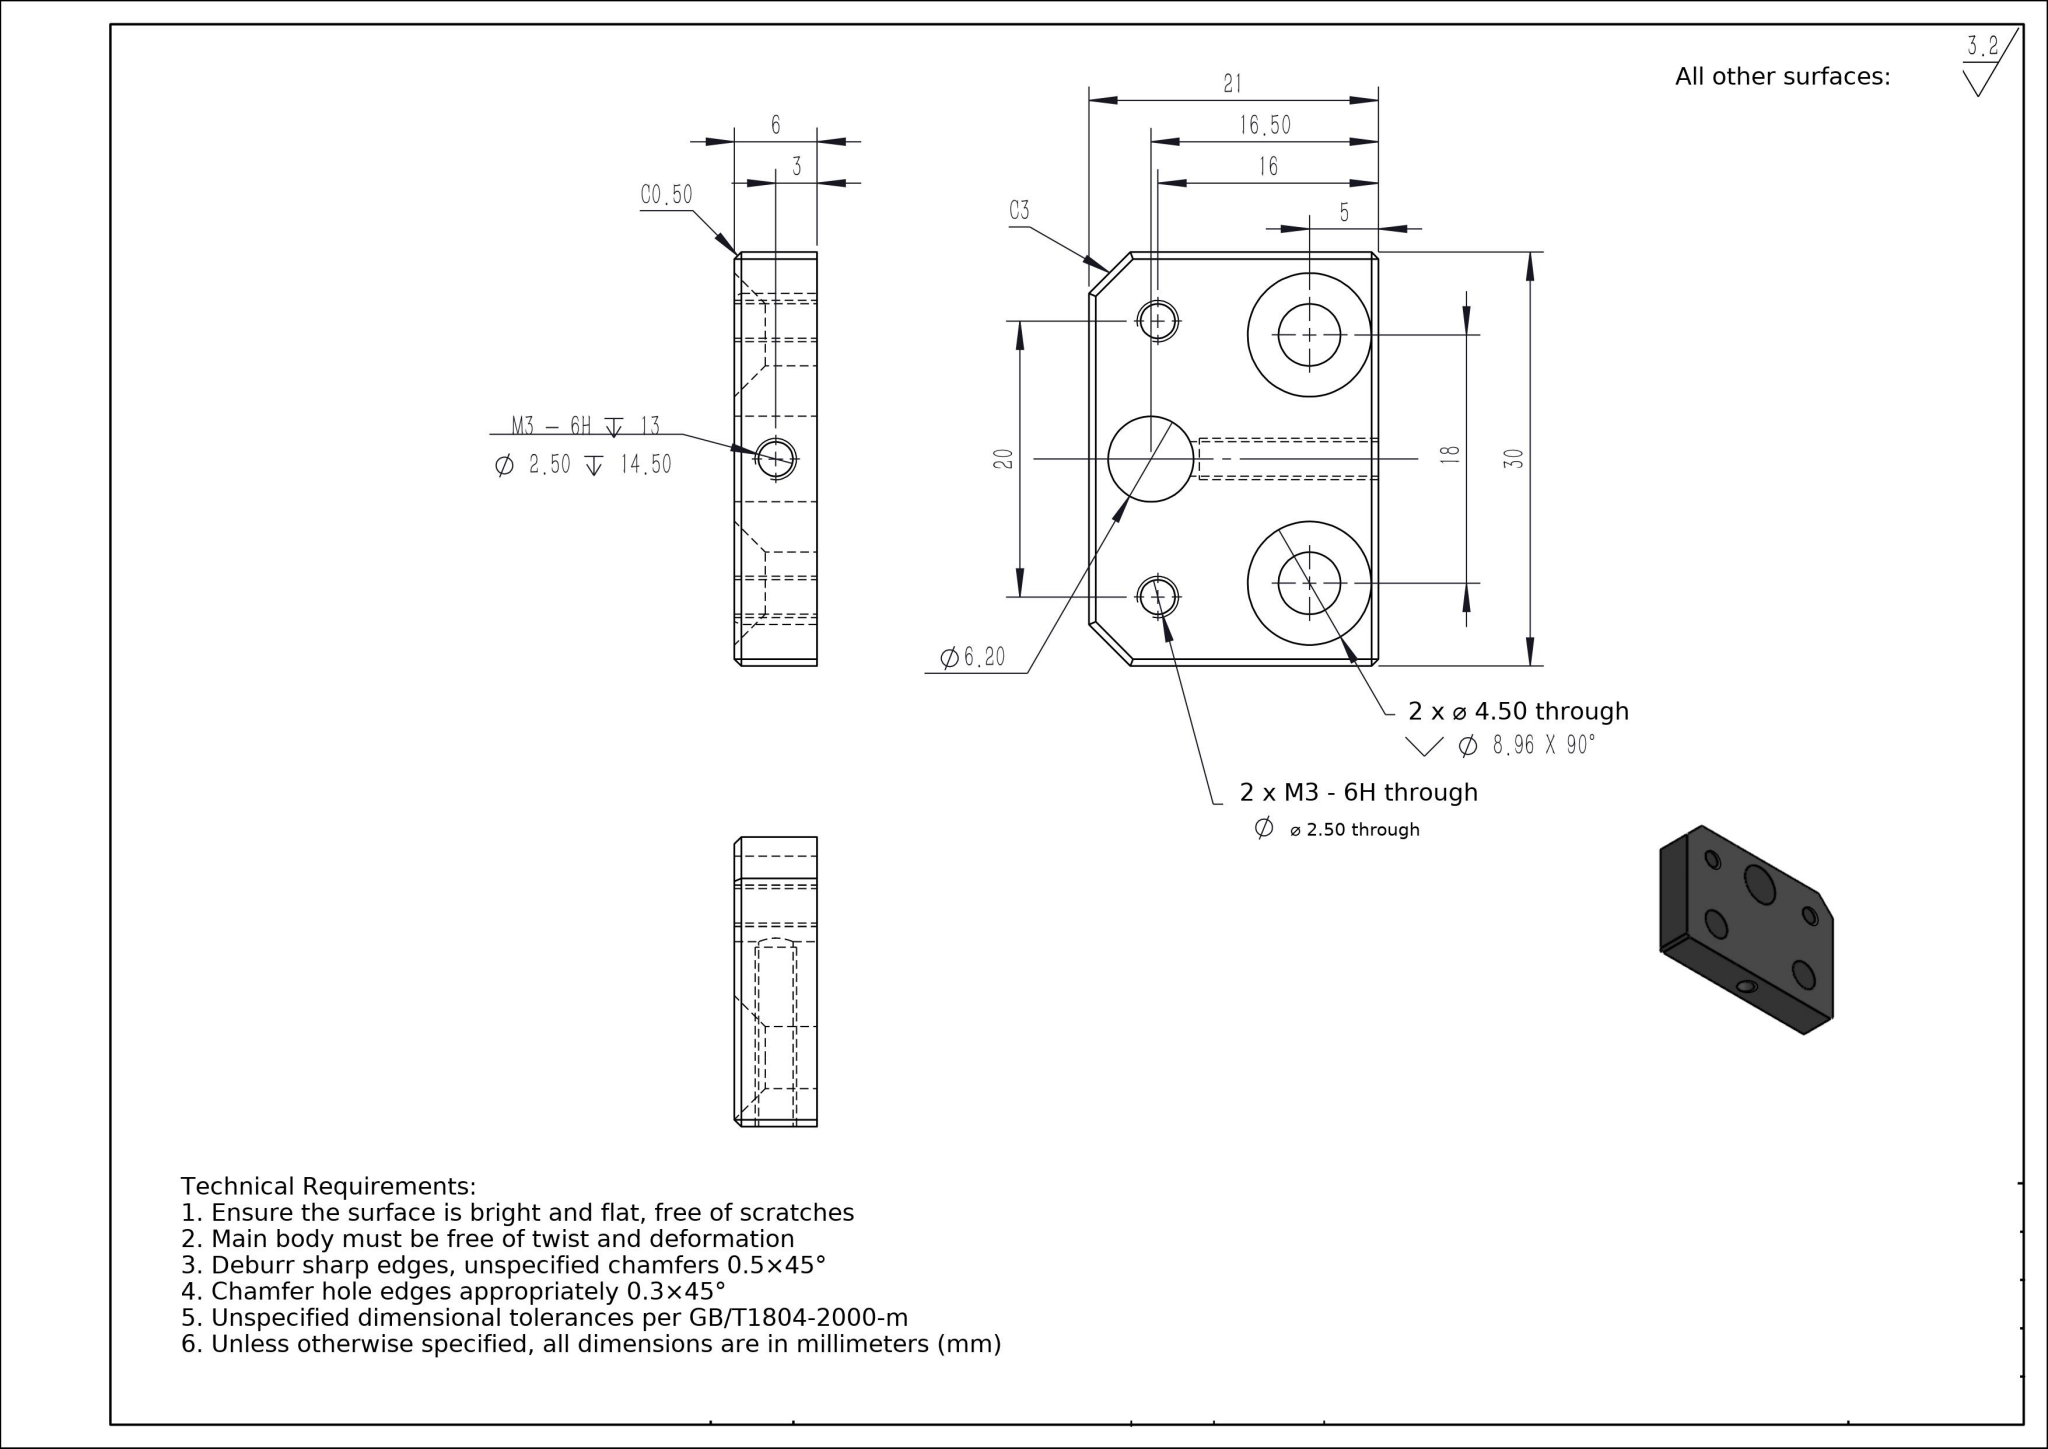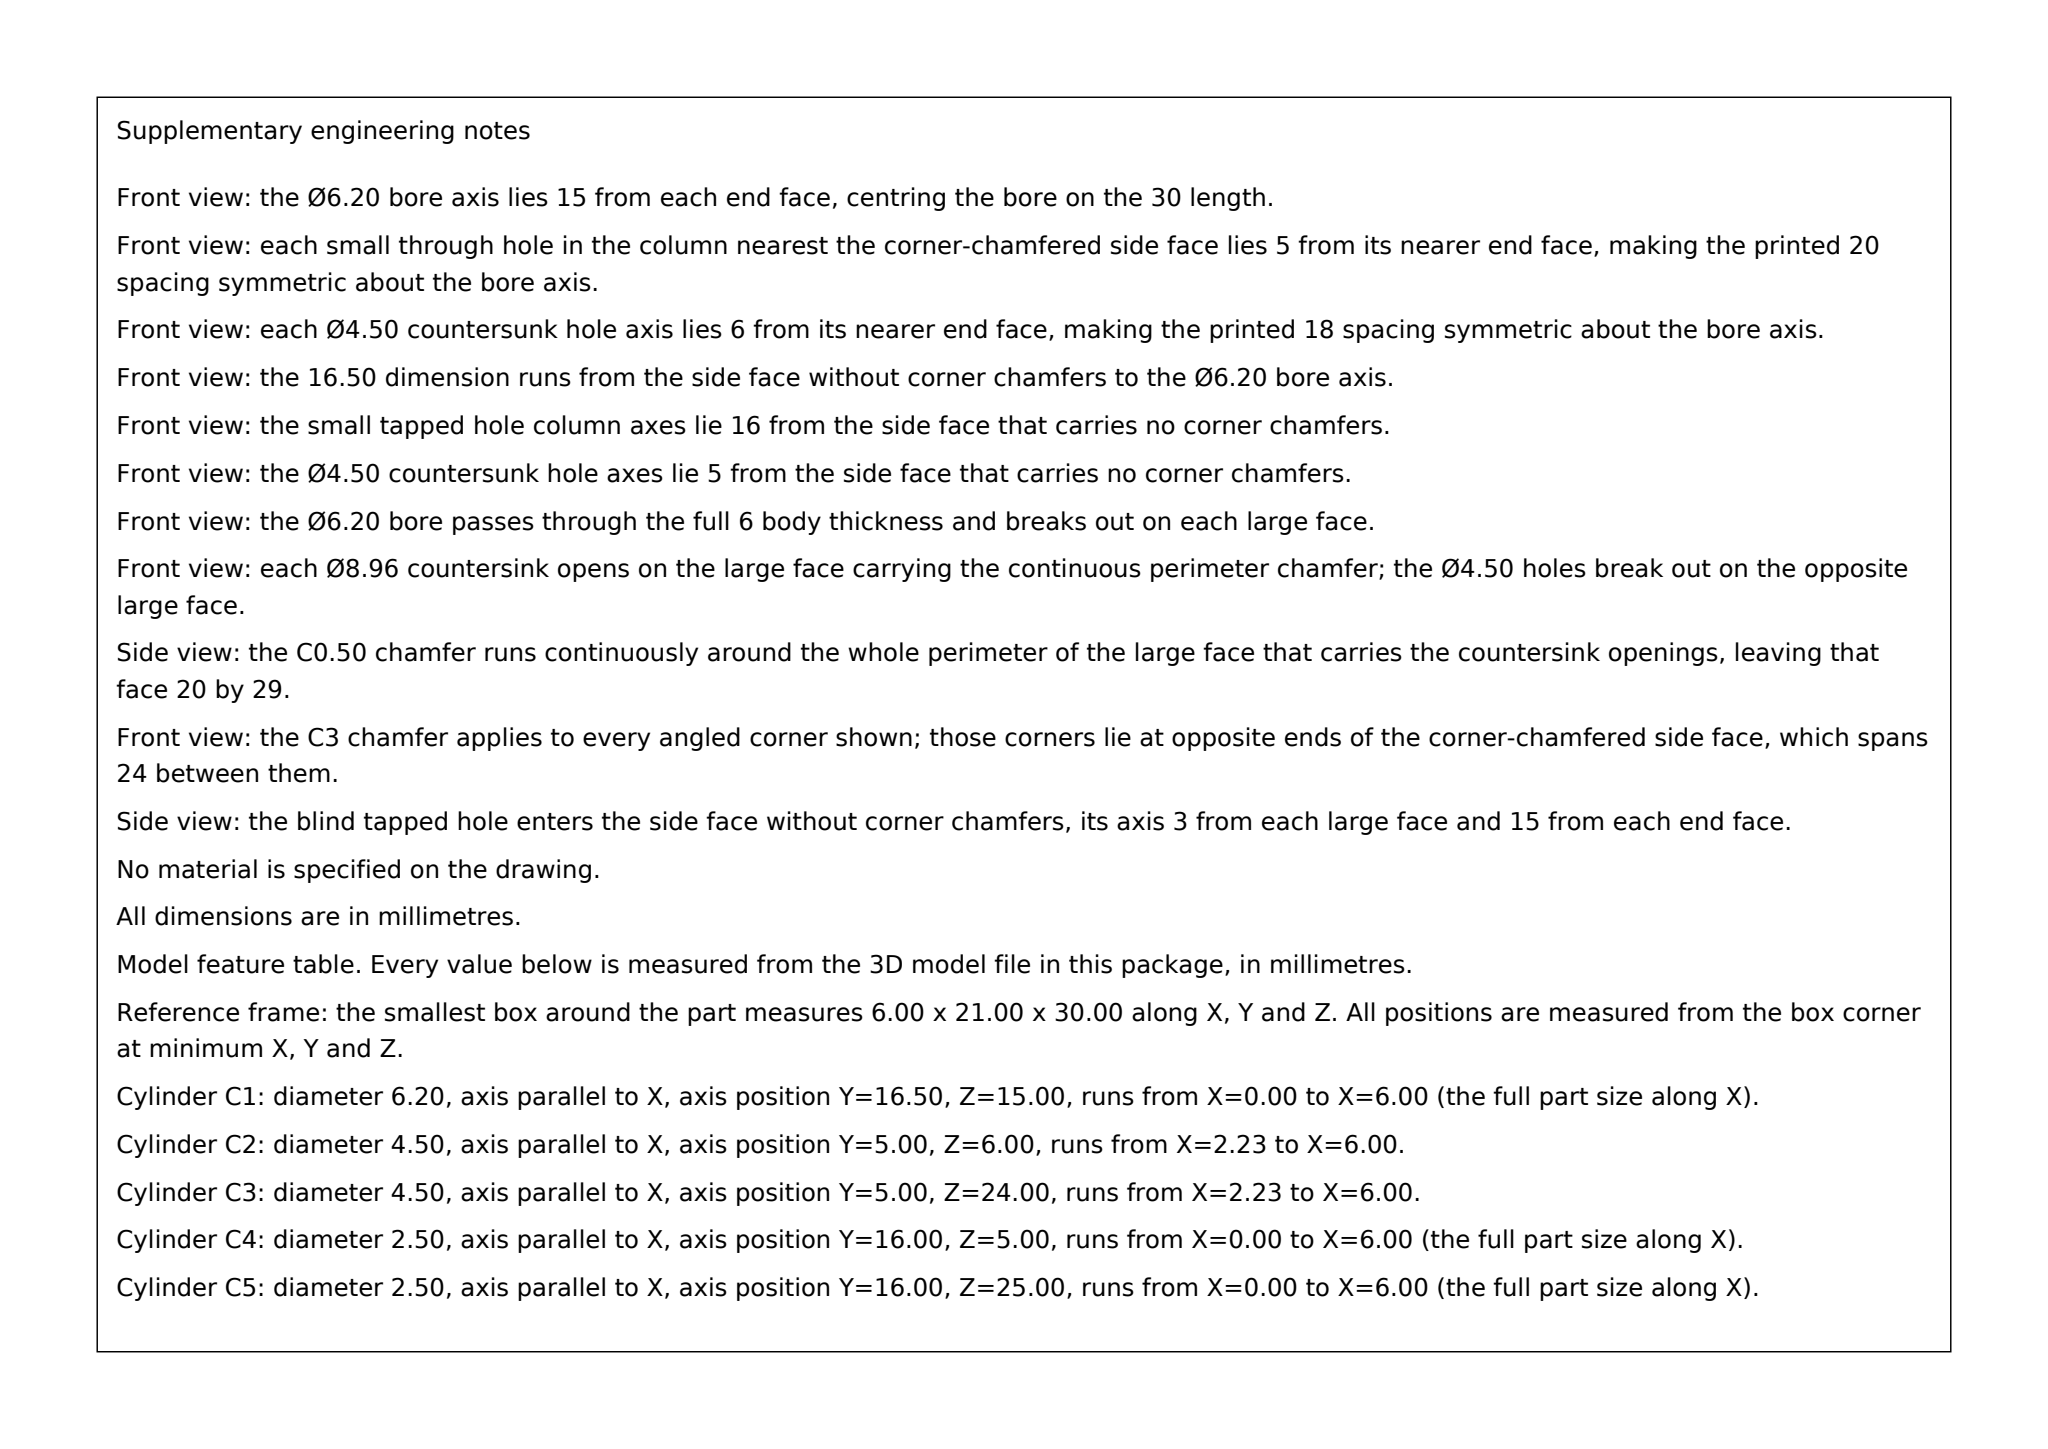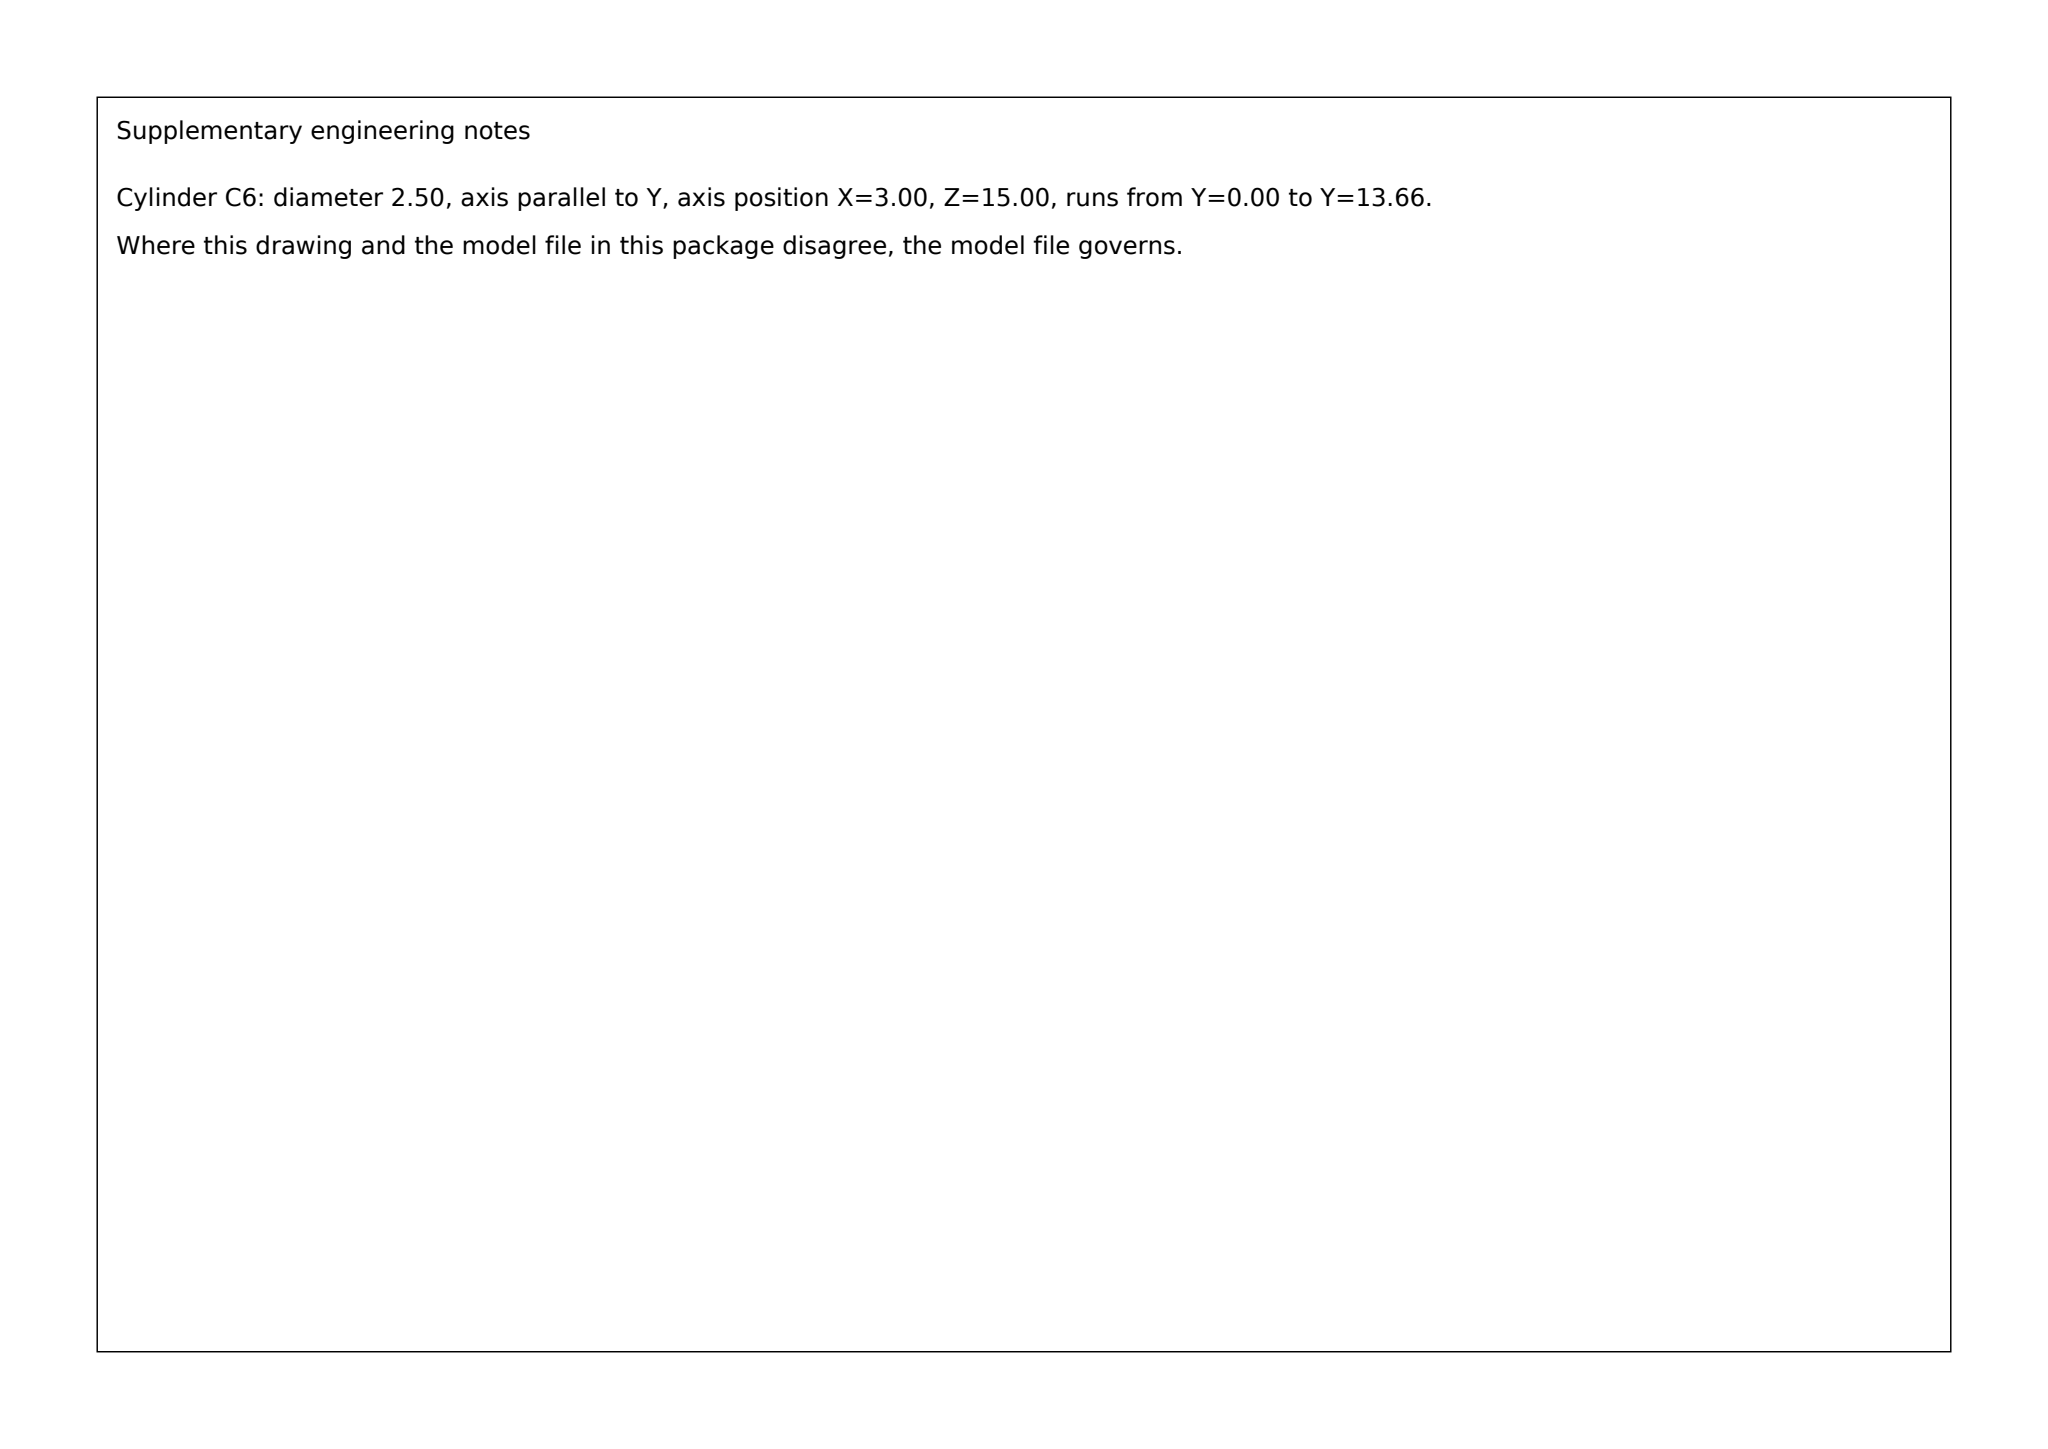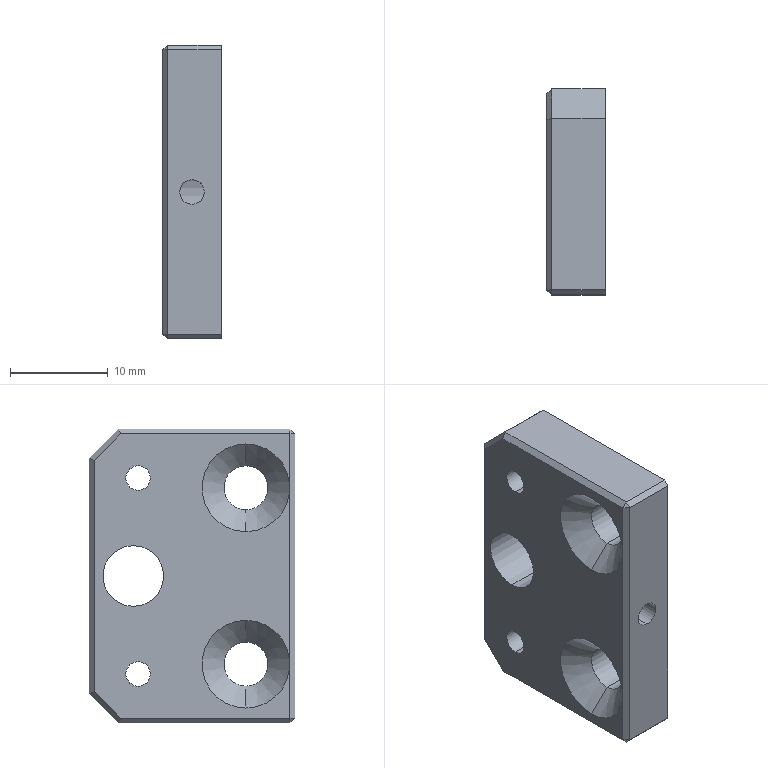Part | SolidWorks | mm | 1 solid | 34 faces | box 6 x 21 x 30 mm | volume 3122 mm3 | plane 18 | cylinder 12 | cone 4 | commonest cylinder face diameters 2.5 x6 4.5 x4 6.2 x2
Drawing notes:
Ø6.20 THRU 6 THK, CL 15 FROM BOTTOM | from the solid: cyl dia 6.2 axis x, len 6.0 = full thk, at y=16.5, z=15.0
Ø2.50 CROSS HOLE DP 13.66, CL 3 FROM FACE, 15 FROM BOTTOM | from the solid: cyl dia 2.5 axis y, len 13.66, at x=3.0, z=15.0
build123d program:
from build123d import *

# Parameters (mm, degrees)
SKETCH1_W                                            = 30
SKETCH1_H                                            = 21
BOSS_EXTRUDE1_DEPTH                                  = 6
CHAMFER1_SIZE                                        = 3
CHAMFER2_SIZE                                        = 0.5
COUNTERSUNK_HOLE_FOR_M4_HEXAGON_COUNTERS_D           = 4.5
COUNTERSUNK_HOLE_FOR_M4_HEXAGON_COUNTERS_CSINK_D     = 8.96
COUNTERSUNK_HOLE_FOR_M4_HEXAGON_COUNTERS_CSINK_ANGLE = 90
SKETCH4_R                                            = 3.1
CUT_EXTRUDE1_DEPTH                                   = 15
M3_TAPPED_HOLE1_D                                    = 2.5
M3_TAPPED_HOLE2_D                                    = 2.5
M3_TAPPED_HOLE2_DEPTH                                = 14.5
M3_TAPPED_HOLE2_TIP                                  = 0.7511


with BuildPart() as part:
    # Sketch1 → Boss-Extrude1 (new body)
    with BuildSketch(Plane(origin=(0, 0, 0), x_dir=(0, 0, -1), z_dir=(1, 0, 0))):
        Rectangle(SKETCH1_W, SKETCH1_H)
    extrude(amount=BOSS_EXTRUDE1_DEPTH)

    # Chamfer1
    chamfer1_edges = [part.edges().sort_by_distance(p)[0] for p in [
        (3, 10.5, 15),
        (3, 10.5, -15),
    ]]
    chamfer(chamfer1_edges, length=CHAMFER1_SIZE)

    # Chamfer2
    chamfer2_edges = [part.edges().sort_by_distance(p)[0] for p in [
        (0, -1.5, 15),
        (0, 10.5, 0),
        (0, 9, -13.5),
        (0, 9, 13.5),
        (0, -1.5, -15),
        (0, -10.5, 0),
        (3, -10.5, -15),
        (3, -10.5, 15),
    ]]
    chamfer(chamfer2_edges, length=CHAMFER2_SIZE)

    # Countersunk hole for M4 Hexagon Counters (through all)
    with Locations(Plane.ZY):
        with Locations((9, -5.5), (-9, -5.5)):
            CounterSinkHole(COUNTERSUNK_HOLE_FOR_M4_HEXAGON_COUNTERS_D / 2, COUNTERSUNK_HOLE_FOR_M4_HEXAGON_COUNTERS_CSINK_D / 2, counter_sink_angle=COUNTERSUNK_HOLE_FOR_M4_HEXAGON_COUNTERS_CSINK_ANGLE)

    # Sketch4 → Cut-Extrude1 (cut)
    with BuildSketch(Plane.ZY):
        with Locations((0, 6)):
            Circle(SKETCH4_R)
    extrude(amount=-CUT_EXTRUDE1_DEPTH, mode=Mode.SUBTRACT)

    # M3 Tapped Hole1 (through all)
    with Locations(Plane(origin=(6, 0, 0), x_dir=(0, 0, -1), z_dir=(1, 0, 0))):
        with Locations((-10, 5.5), (10, 5.5)):
            Hole(M3_TAPPED_HOLE1_D / 2)

    # M3 Tapped Hole2
    with Locations(Plane(origin=(0, -10.5, 0), x_dir=(-1, 0, 0), z_dir=(0, -1, 0))):
        with Locations((-3, 0)):
            Hole(M3_TAPPED_HOLE2_D / 2, depth=M3_TAPPED_HOLE2_DEPTH)
            with Locations((0, 0, -(M3_TAPPED_HOLE2_DEPTH + M3_TAPPED_HOLE2_TIP / 2))):  # 118° drill point
                Cone(0, M3_TAPPED_HOLE2_D / 2, M3_TAPPED_HOLE2_TIP, mode=Mode.SUBTRACT)


solid = part.part